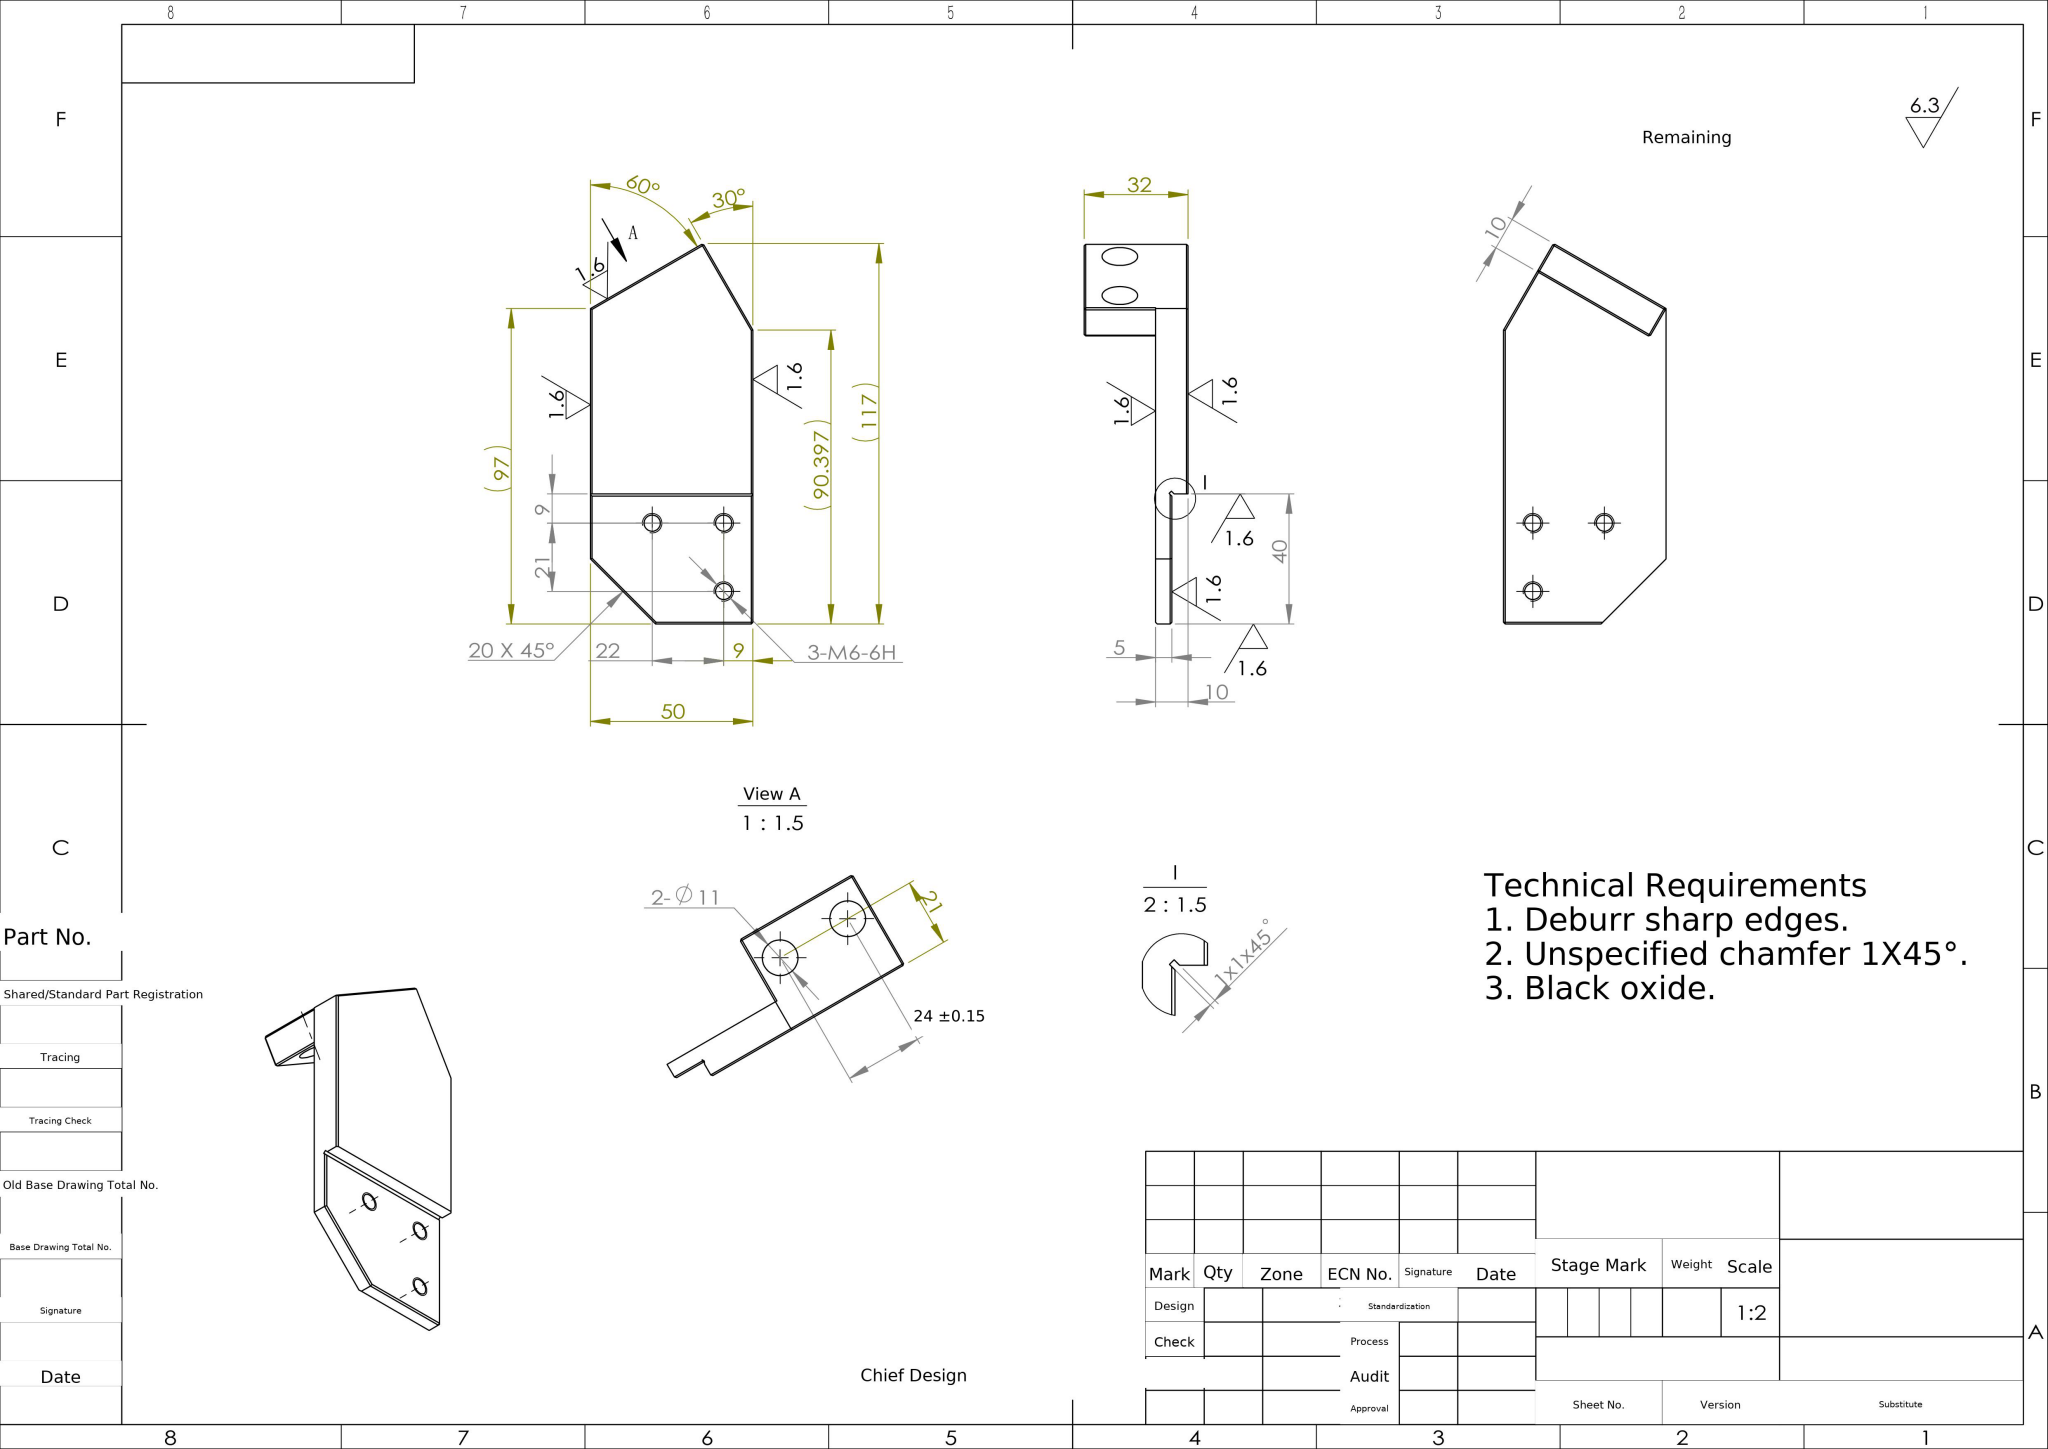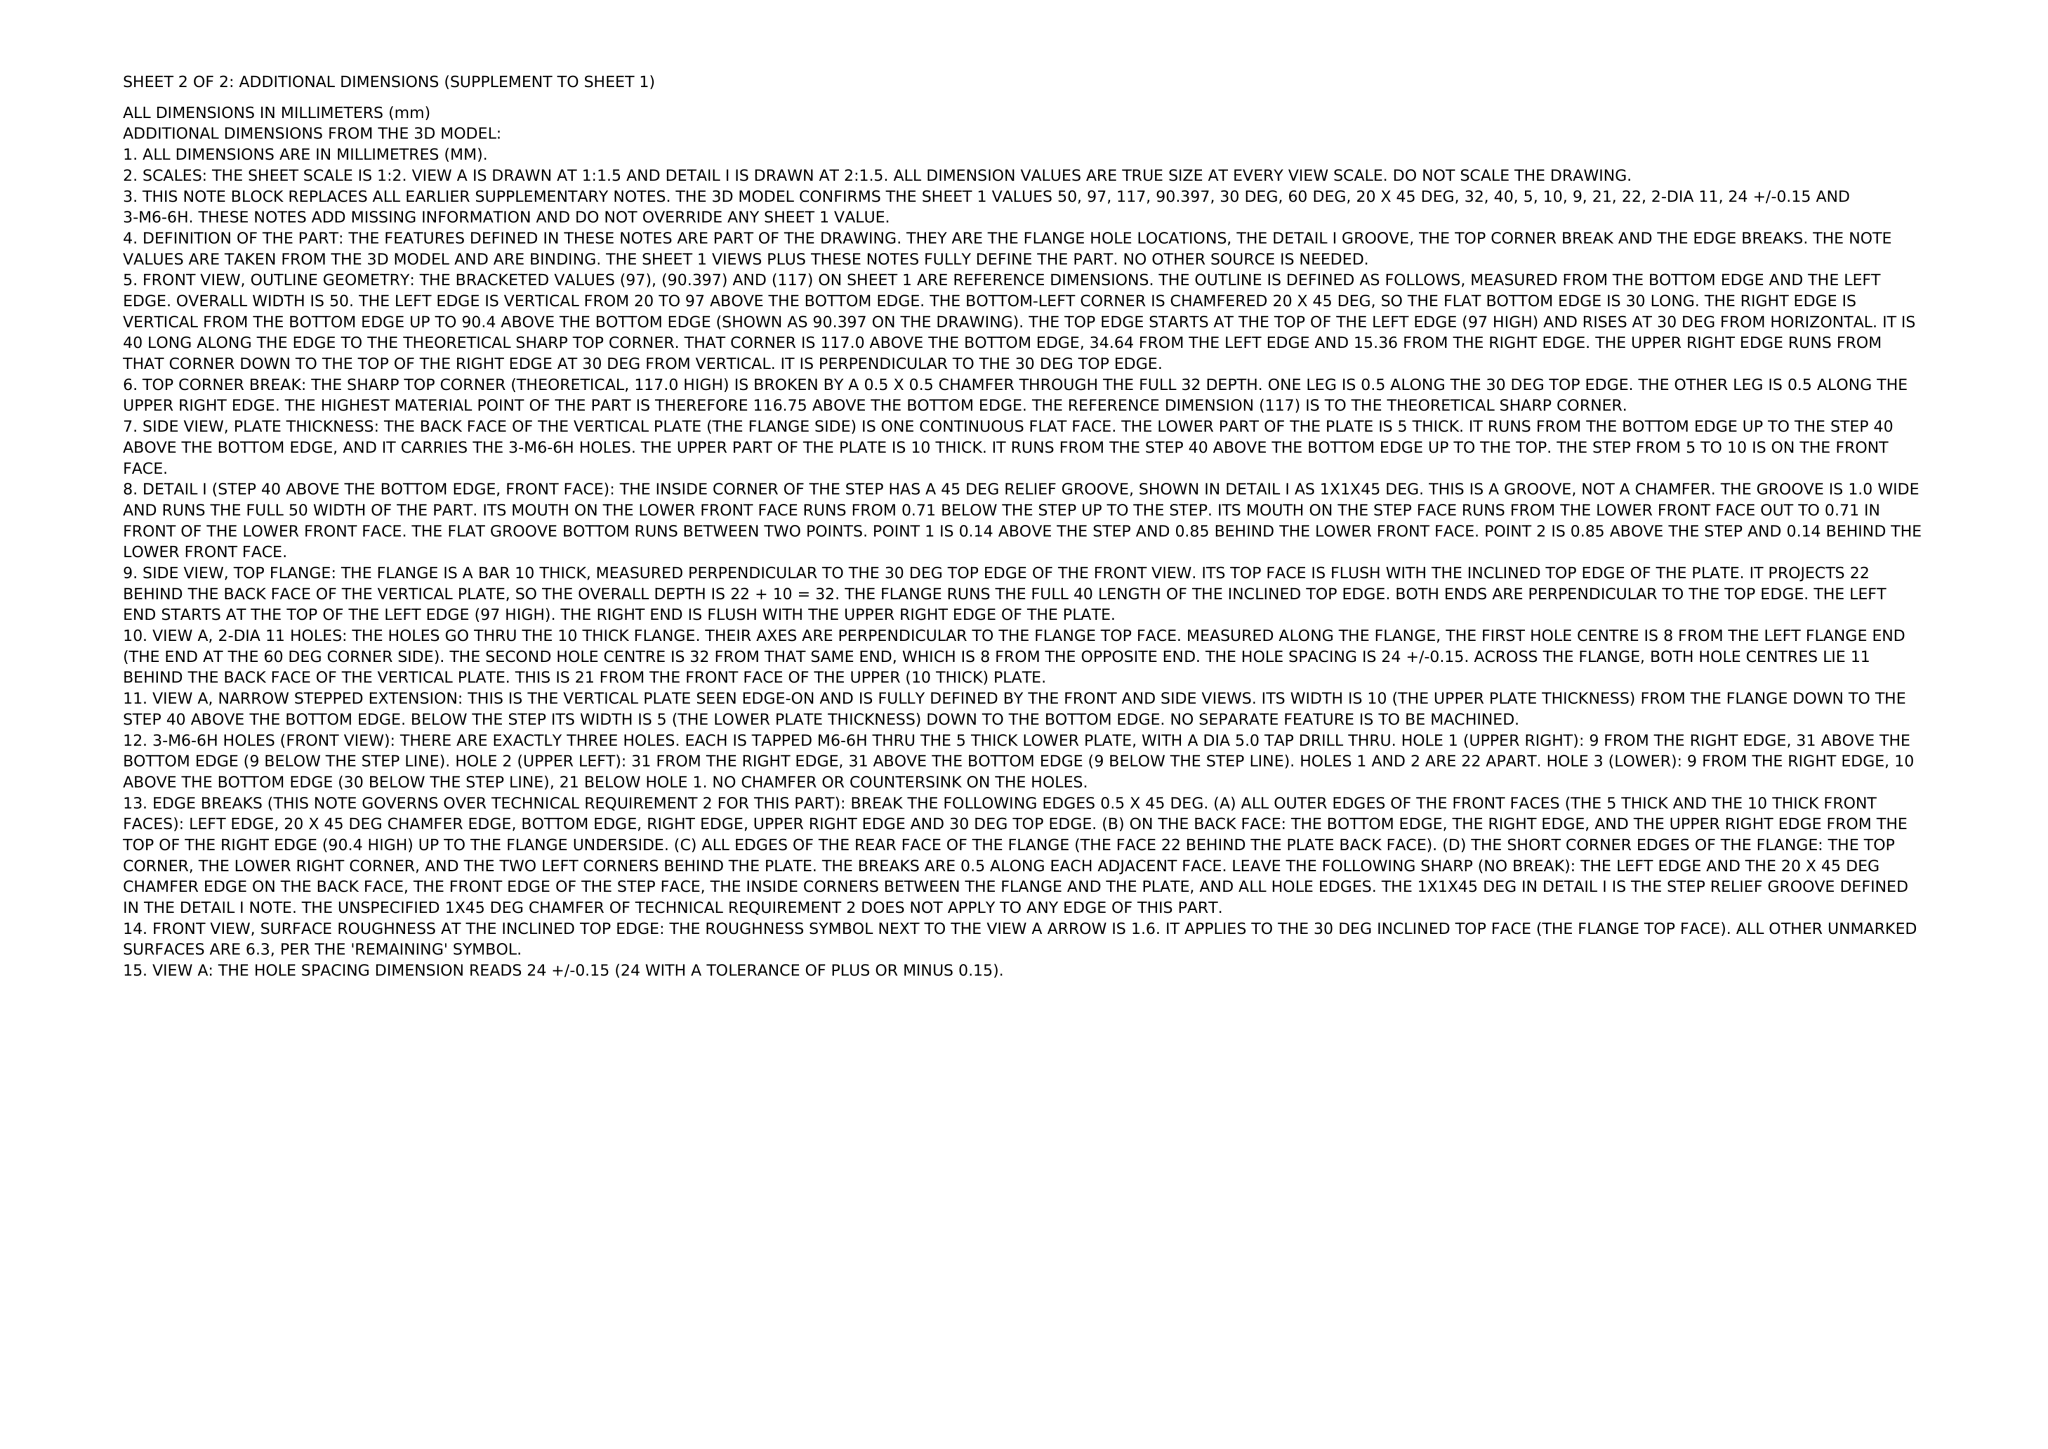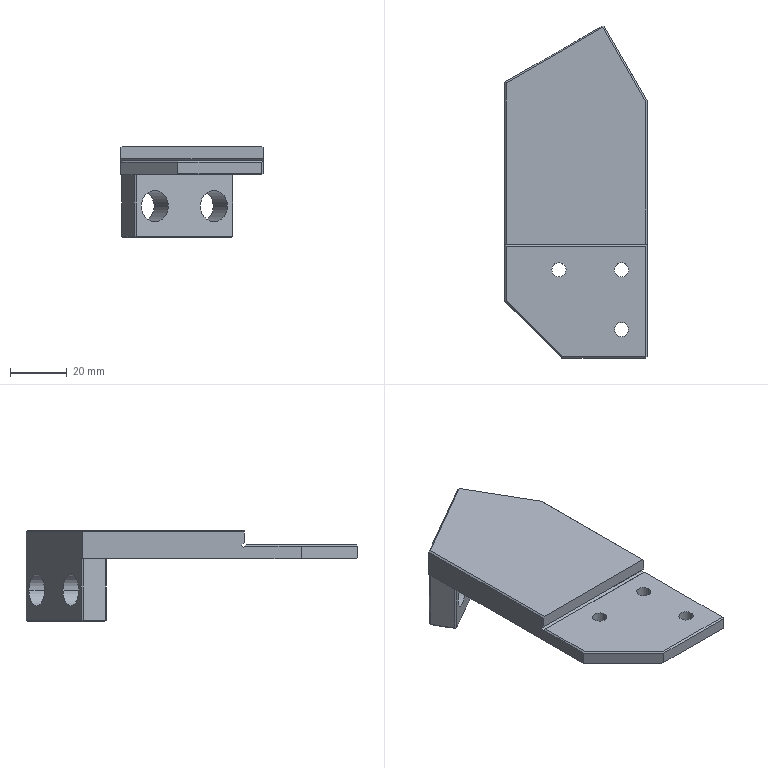Part | NX | mm | Angled Top Gusseted Mounting Bracket | 1 solid | 53 faces | box 50 x 116.75 x 32 mm | volume 48471 mm3 | plane 43 | cylinder 10 | commonest cylinder face diameters 5 x6 11 x4